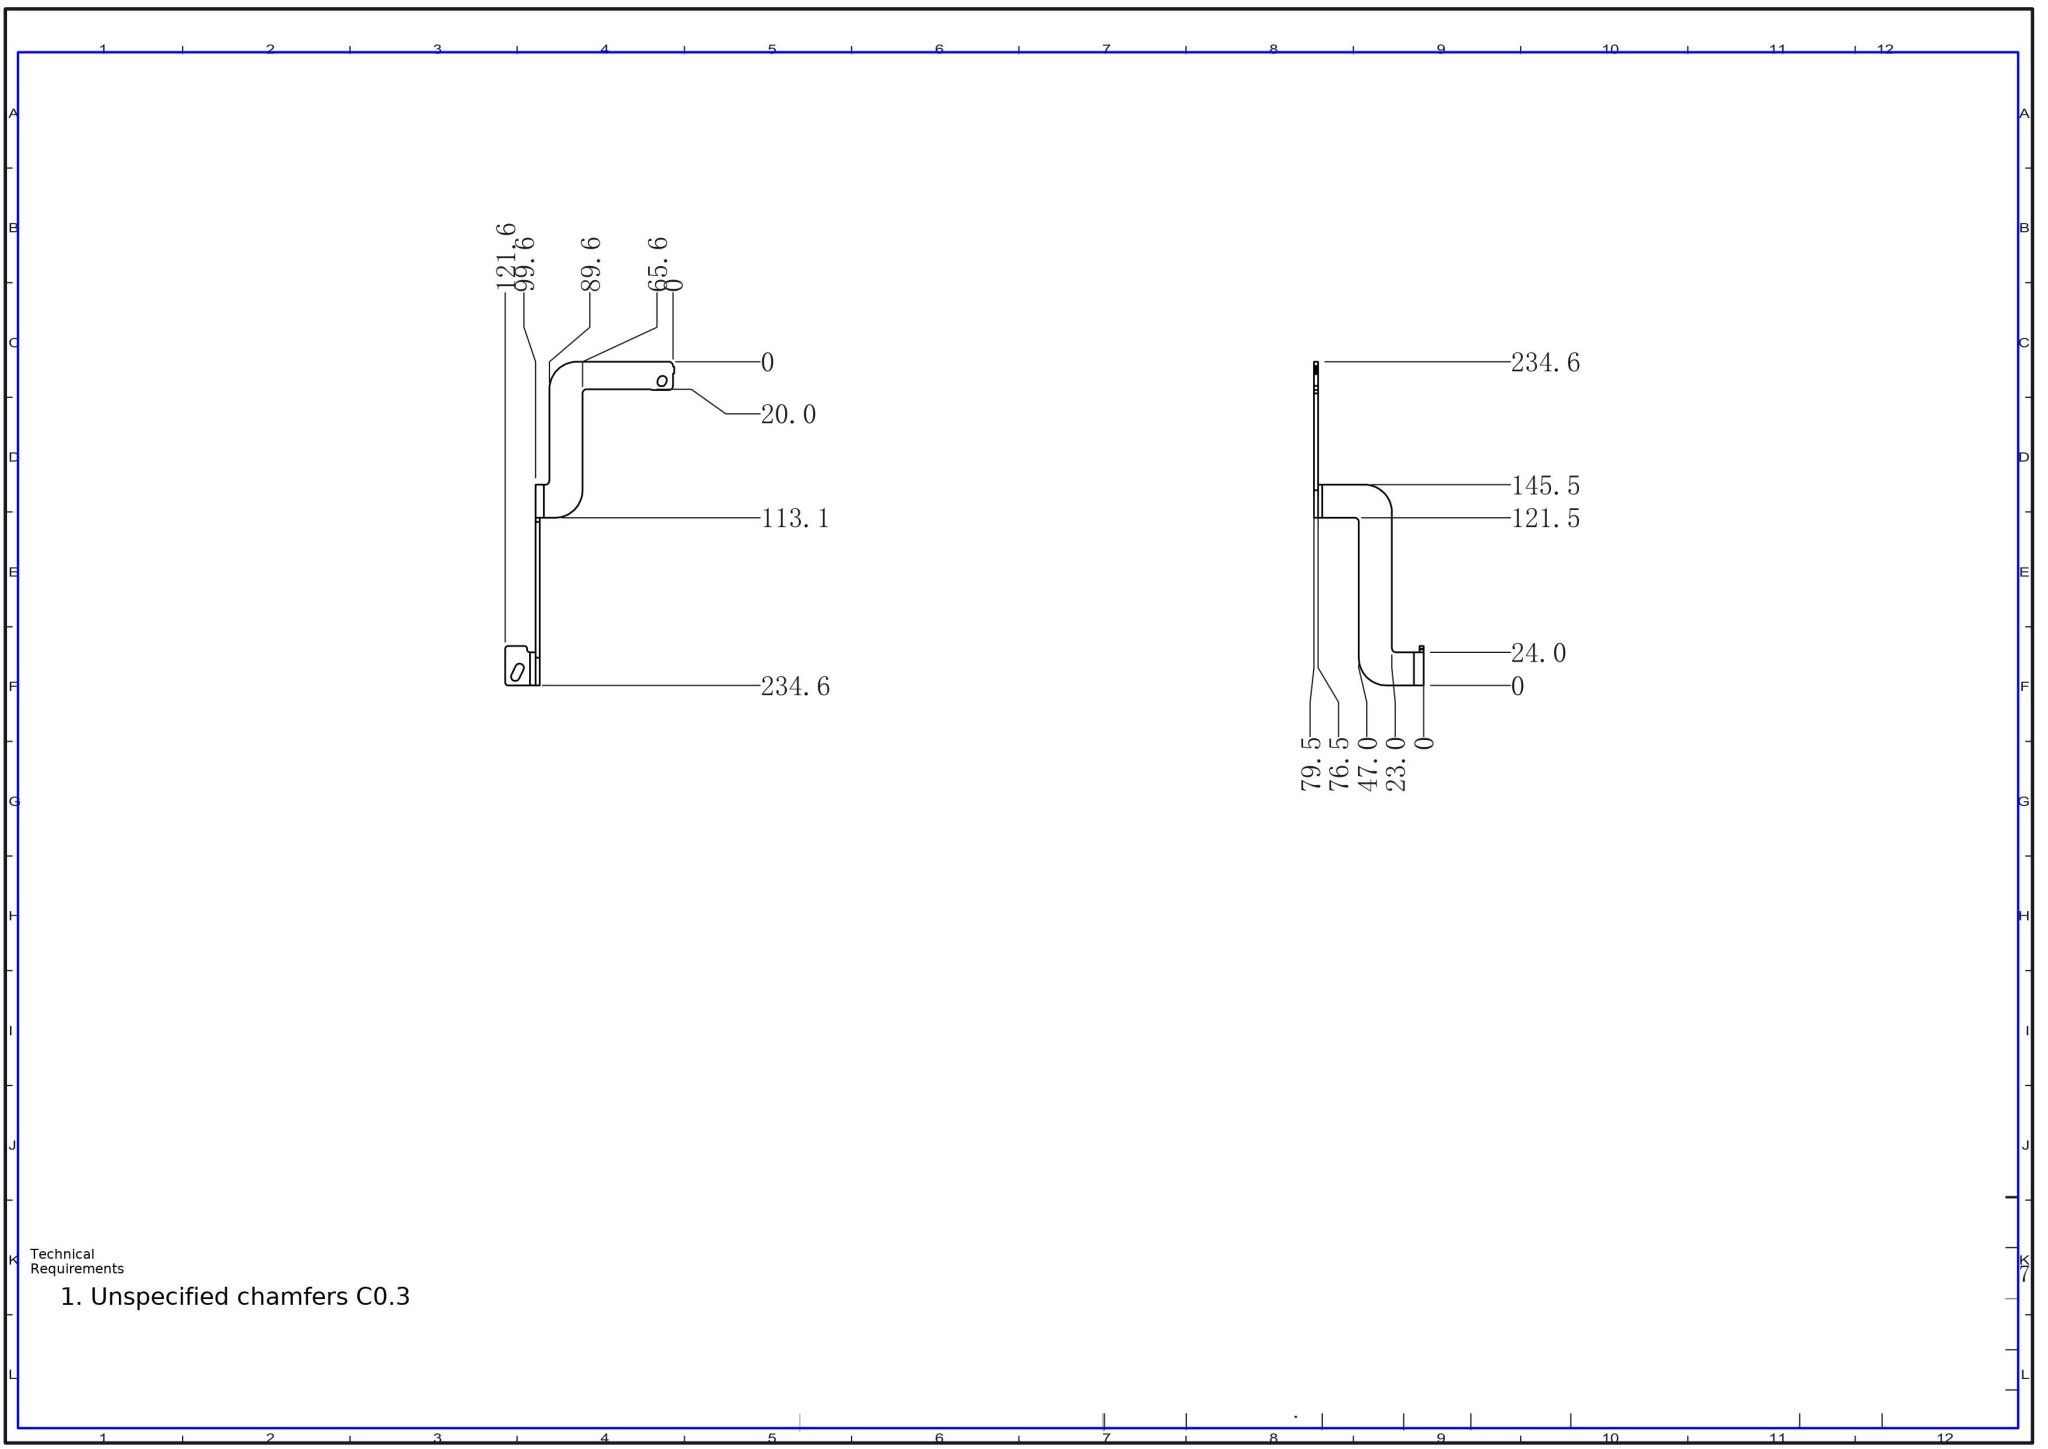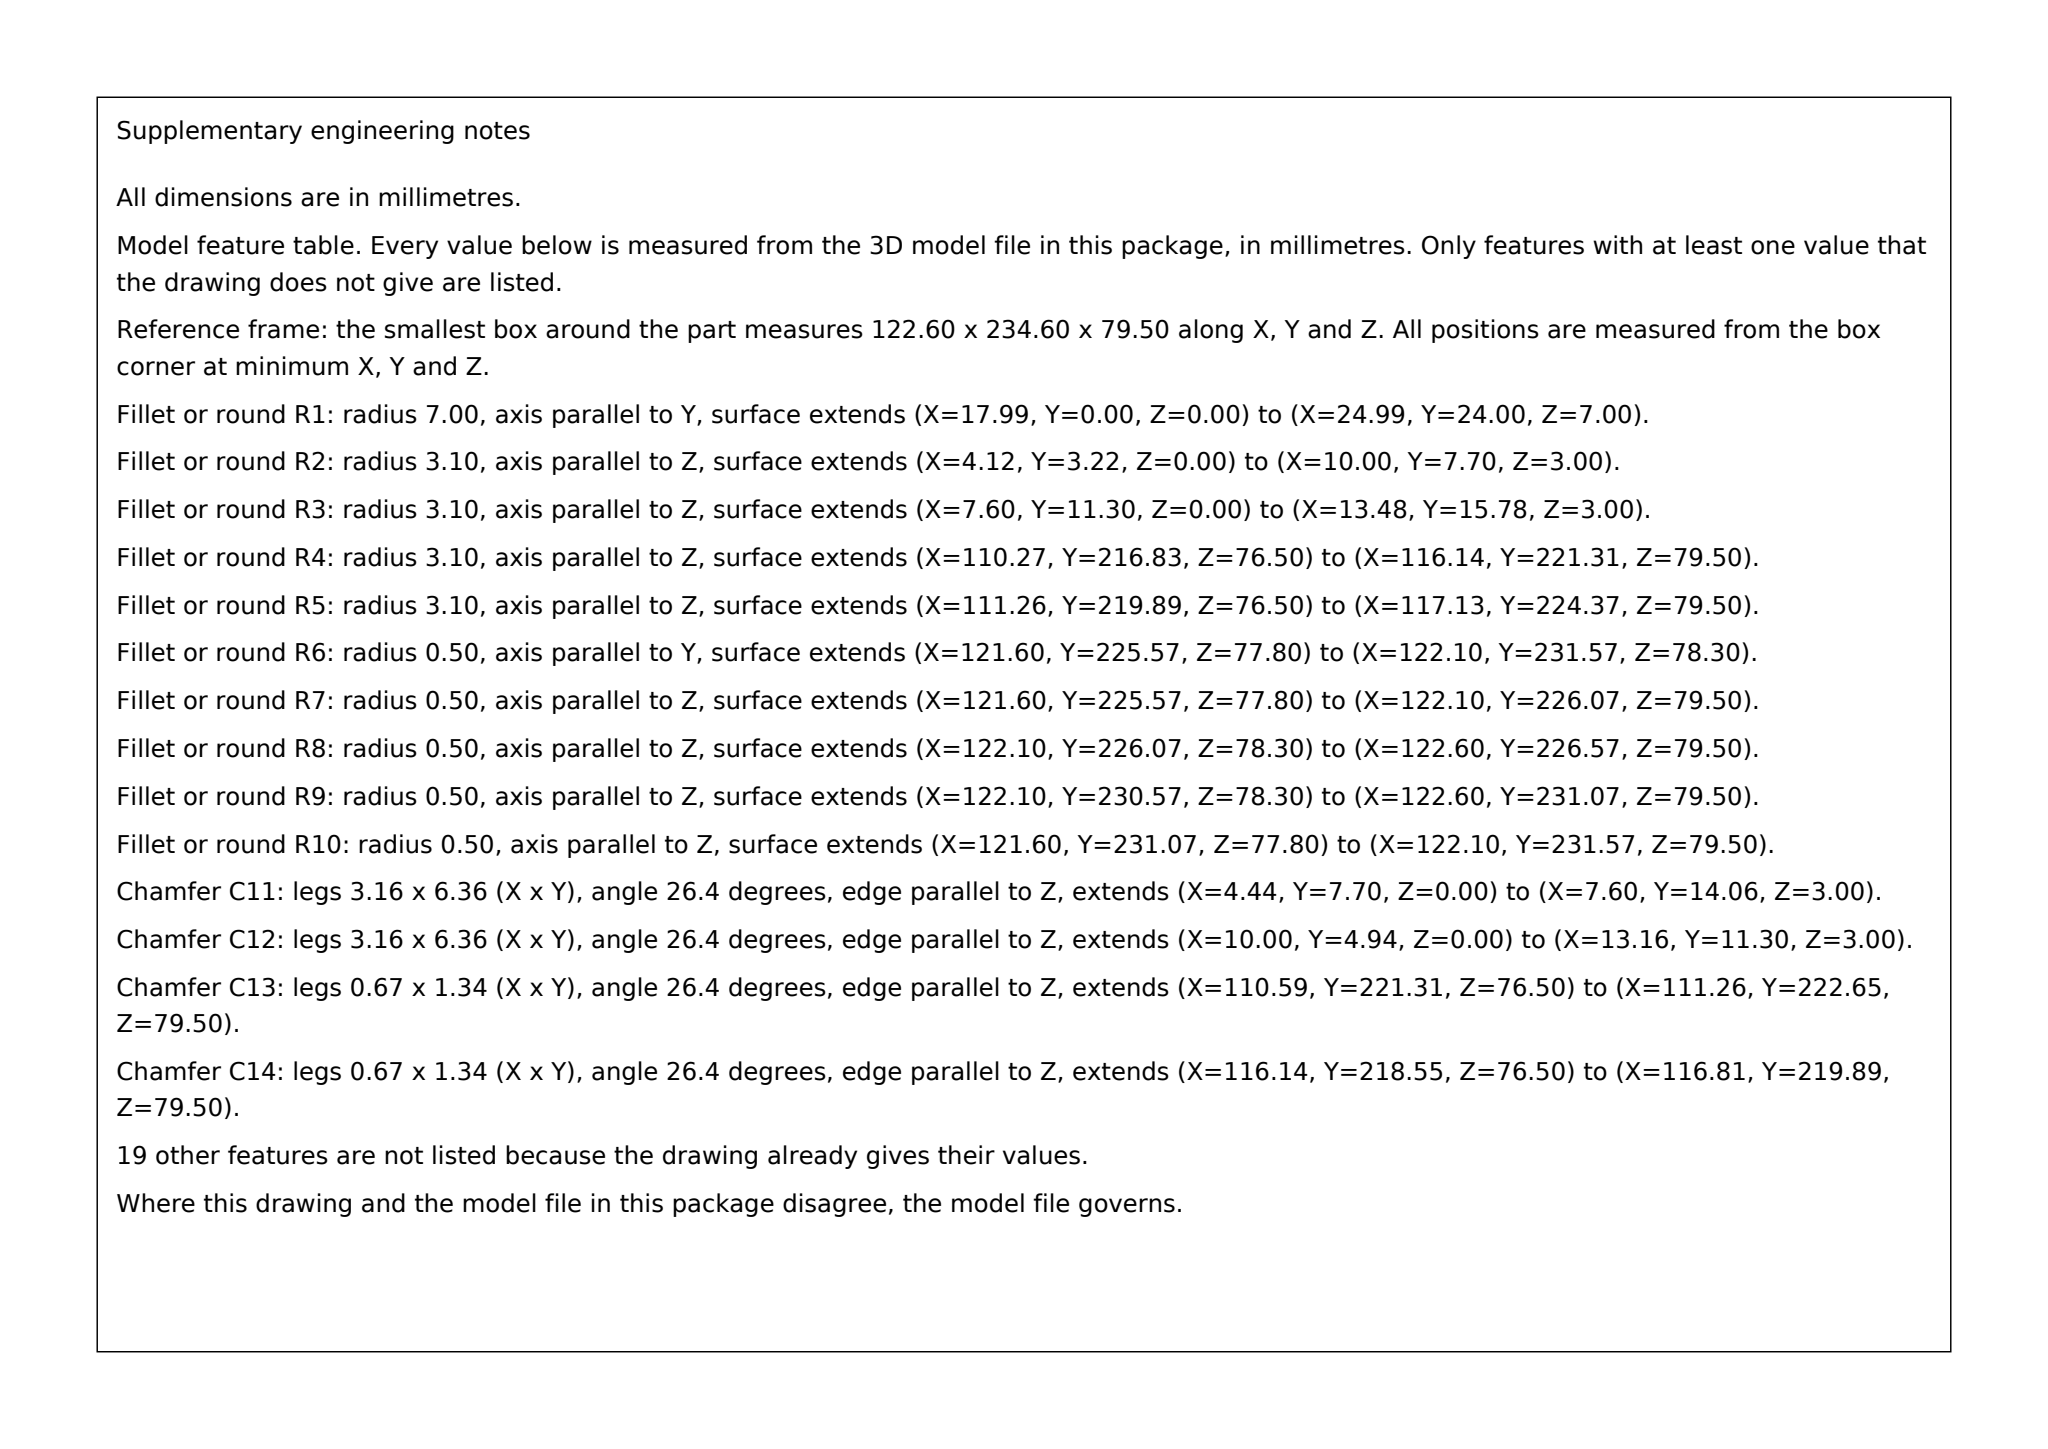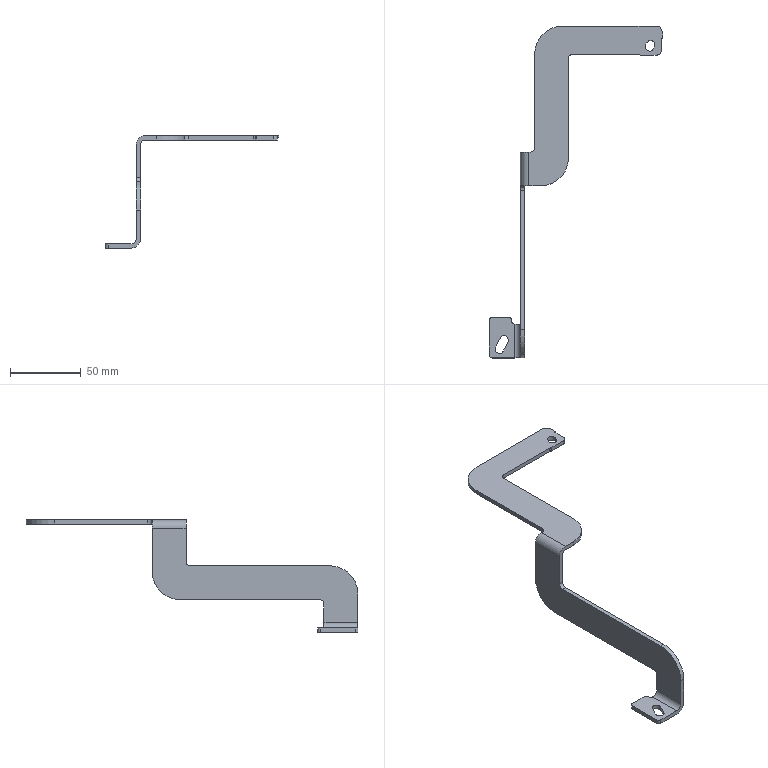Part | SolidWorks | mm | 1 solid | 58 faces | box 122.6 x 234.6 x 79.5 mm | volume 27211 mm3 | cylinder 31 | plane 27 | commonest cylinder face diameters 6 x7 6.2 x6 4 x6 1 x5 40 x4 14 x1 8 x1 12 x1